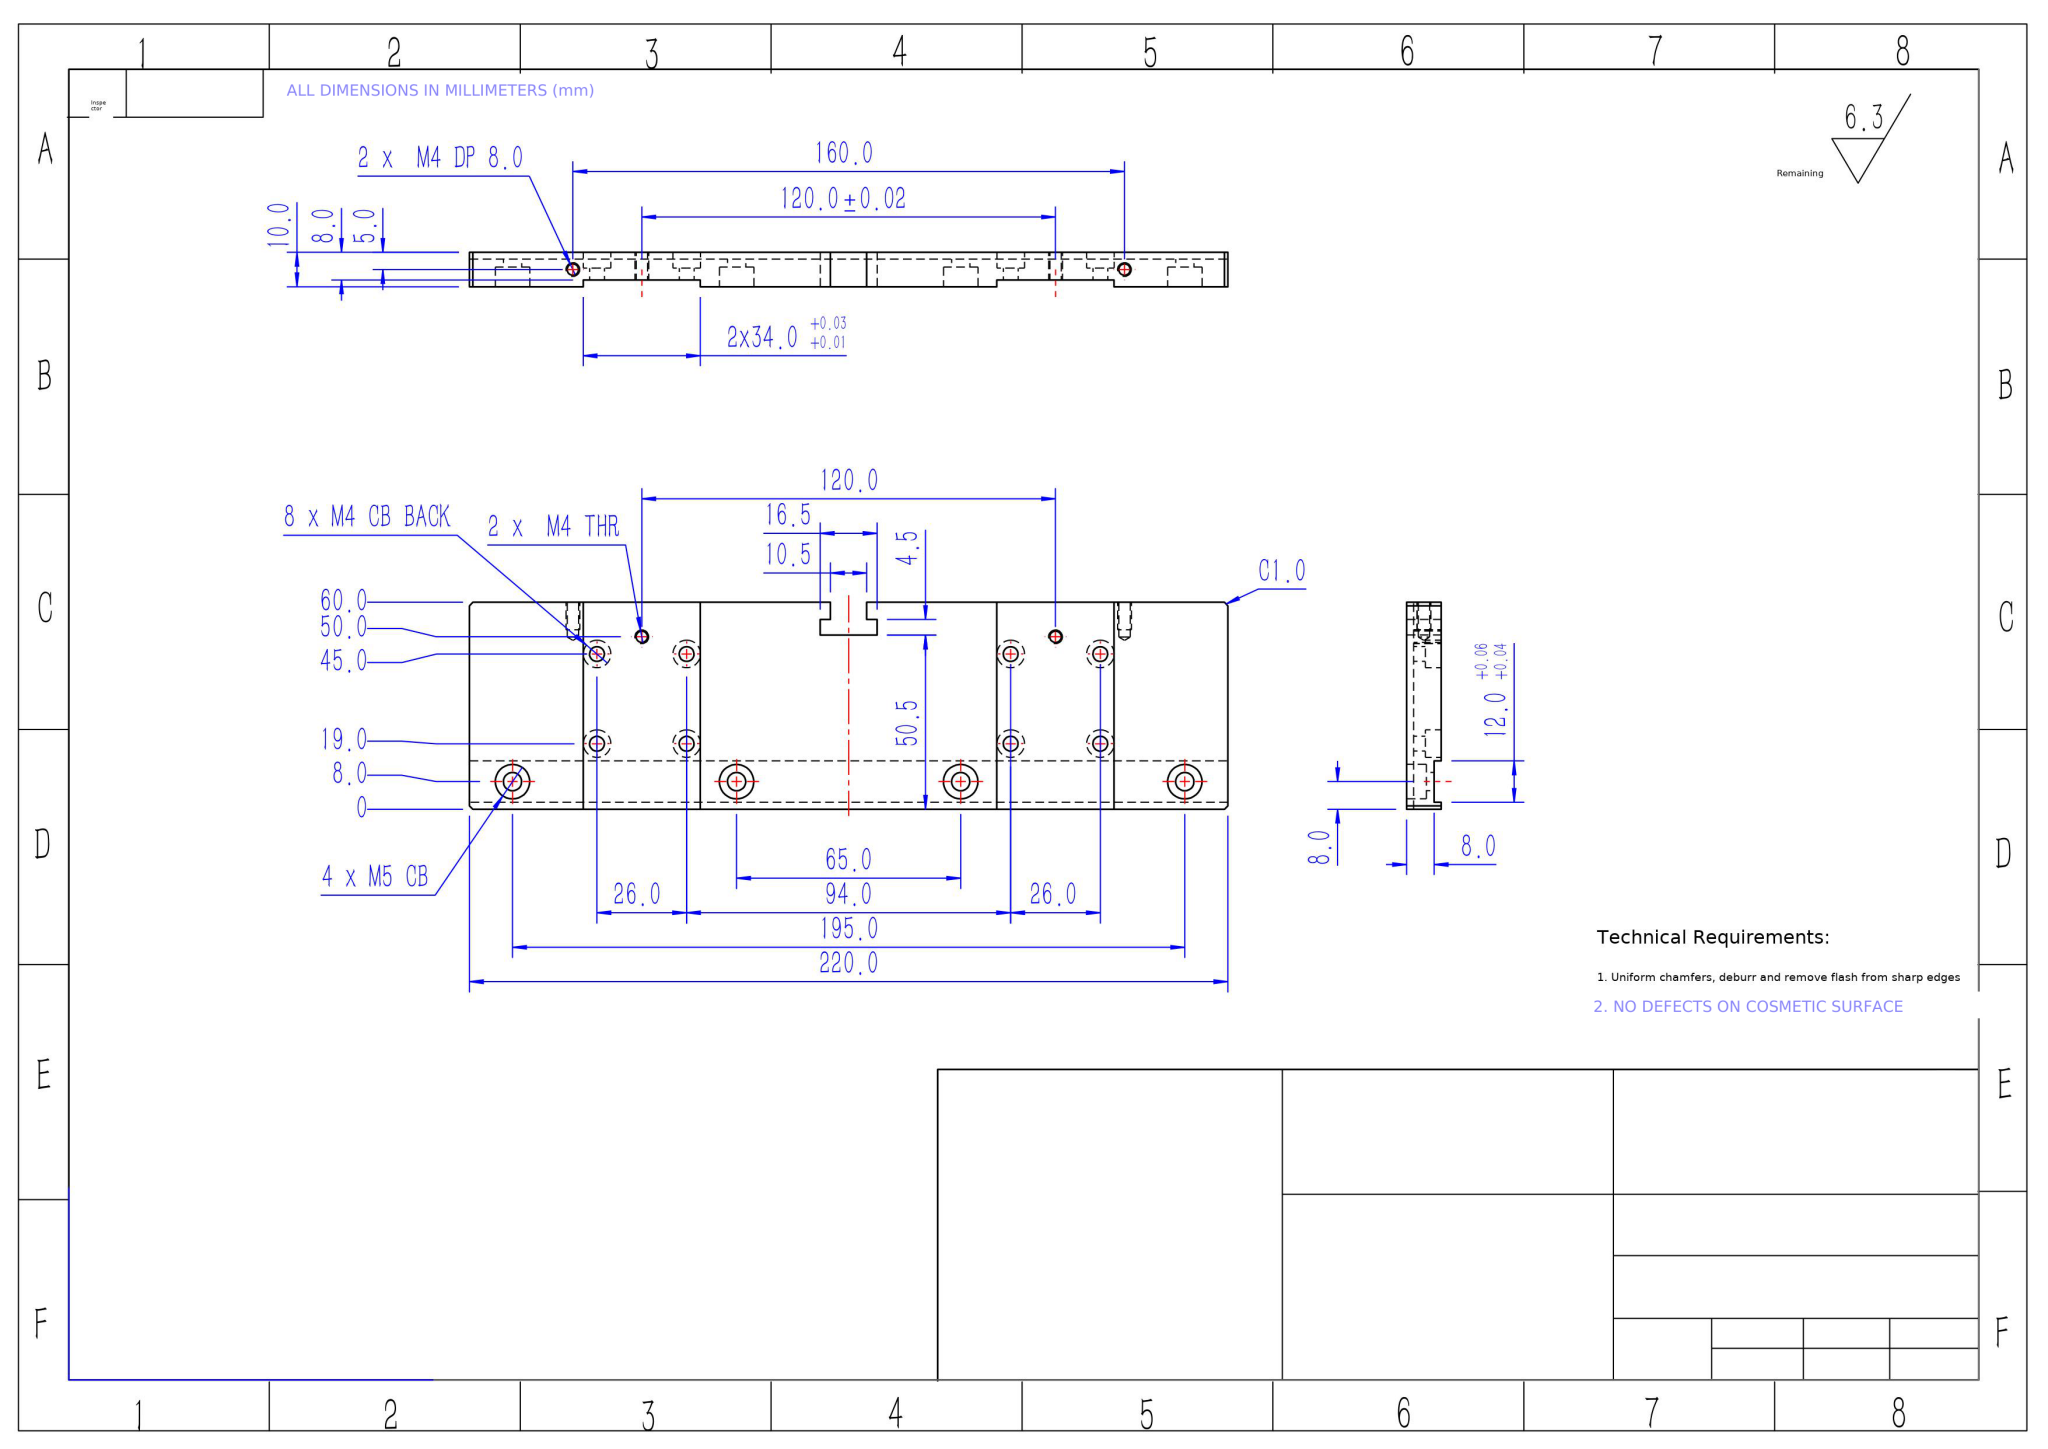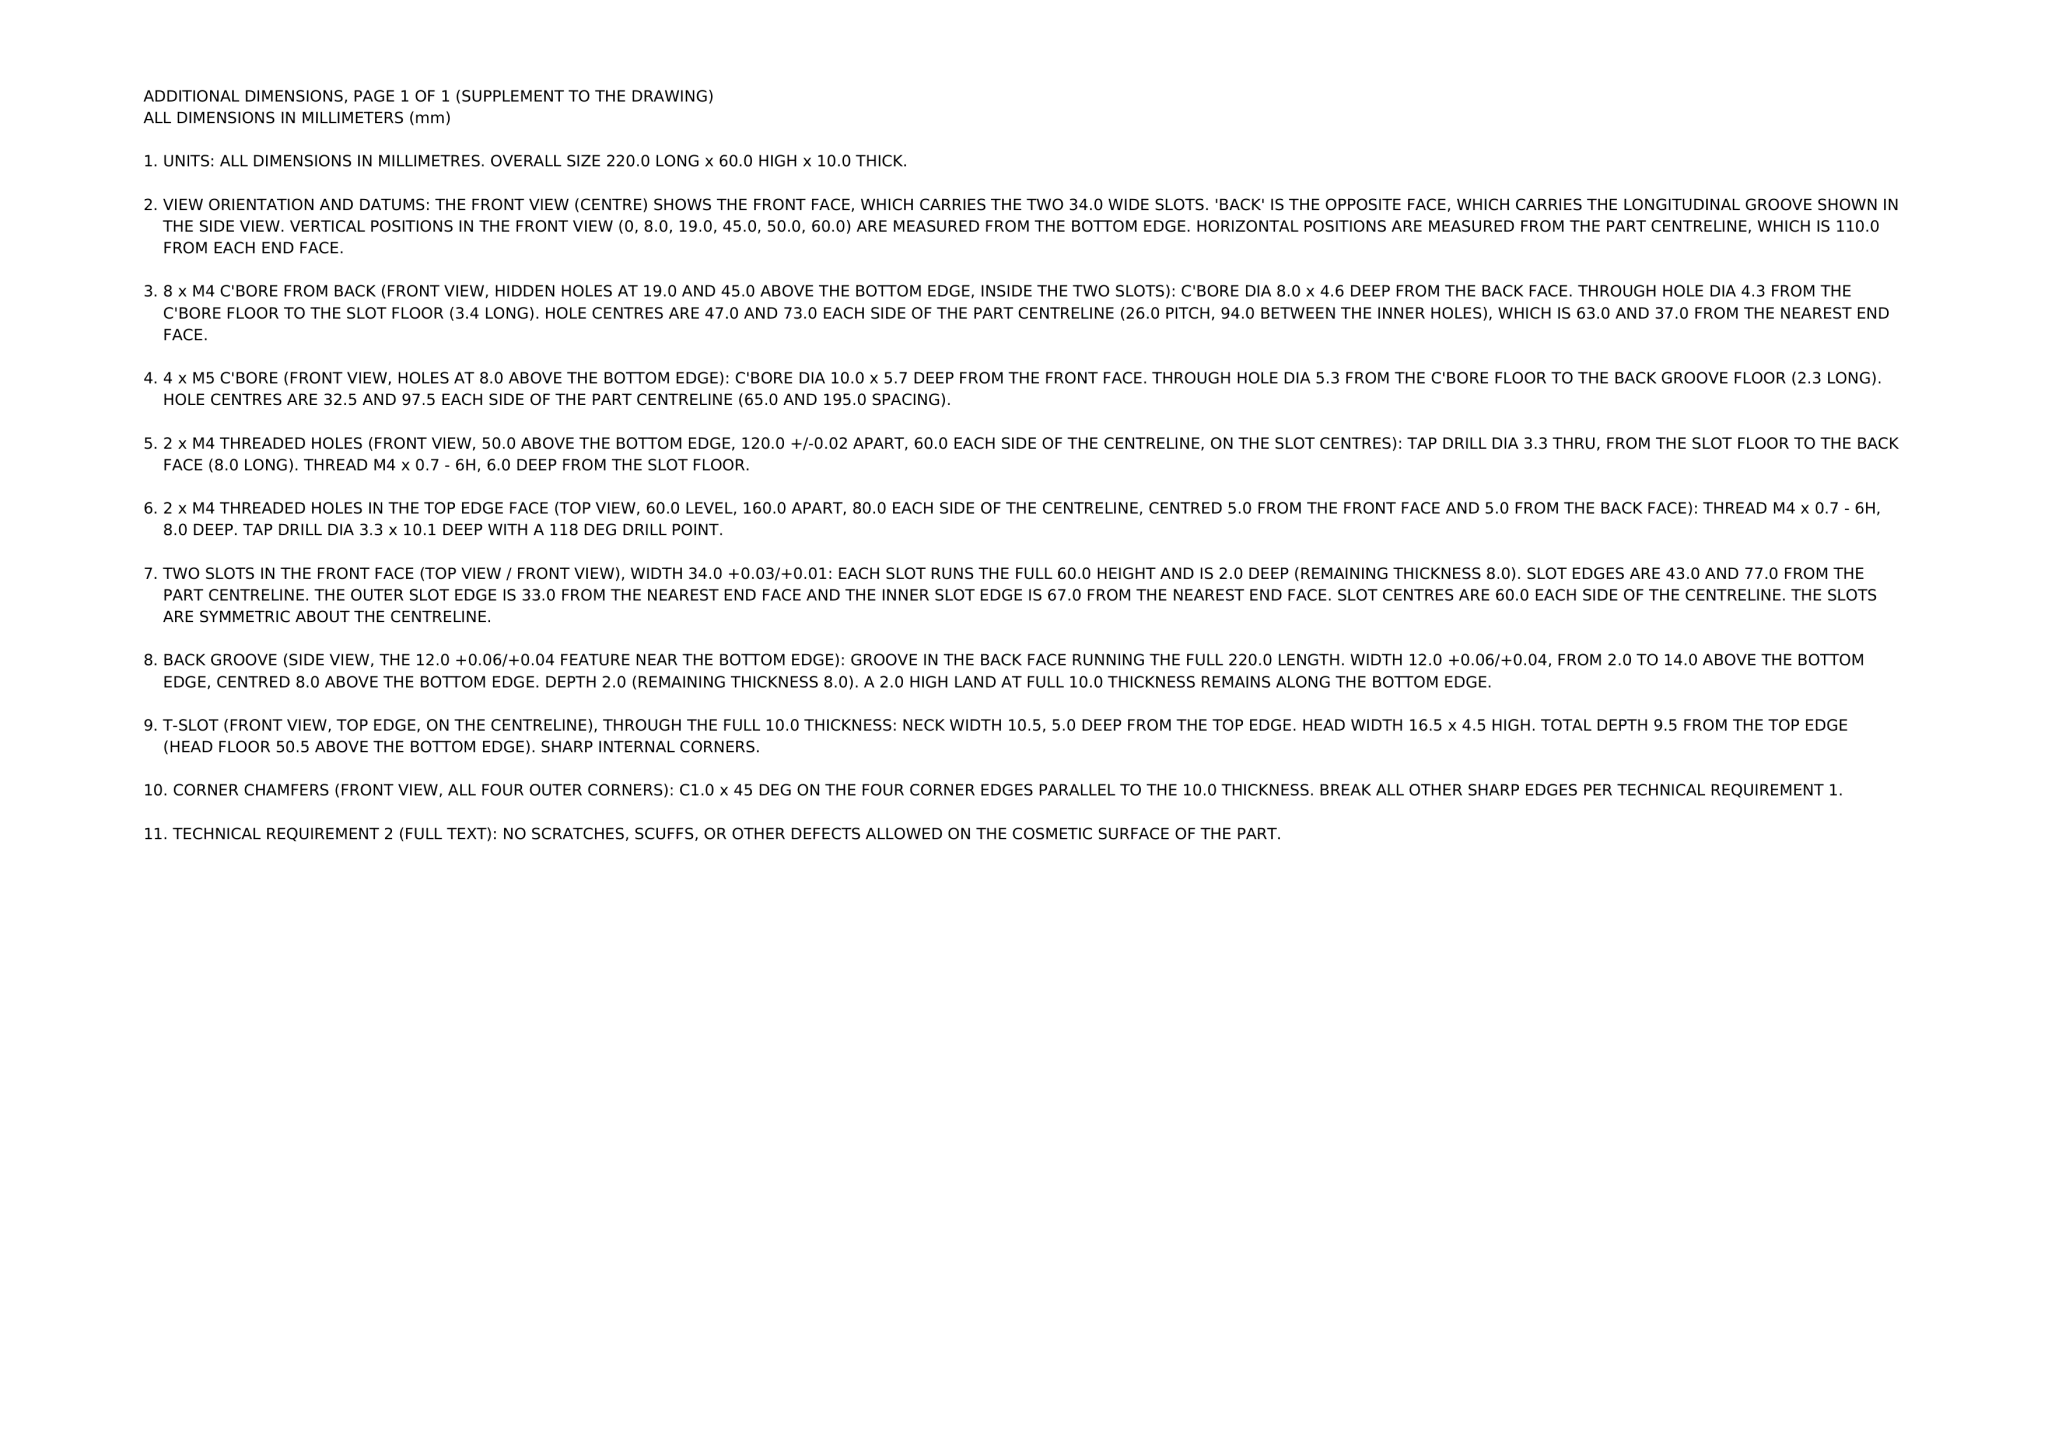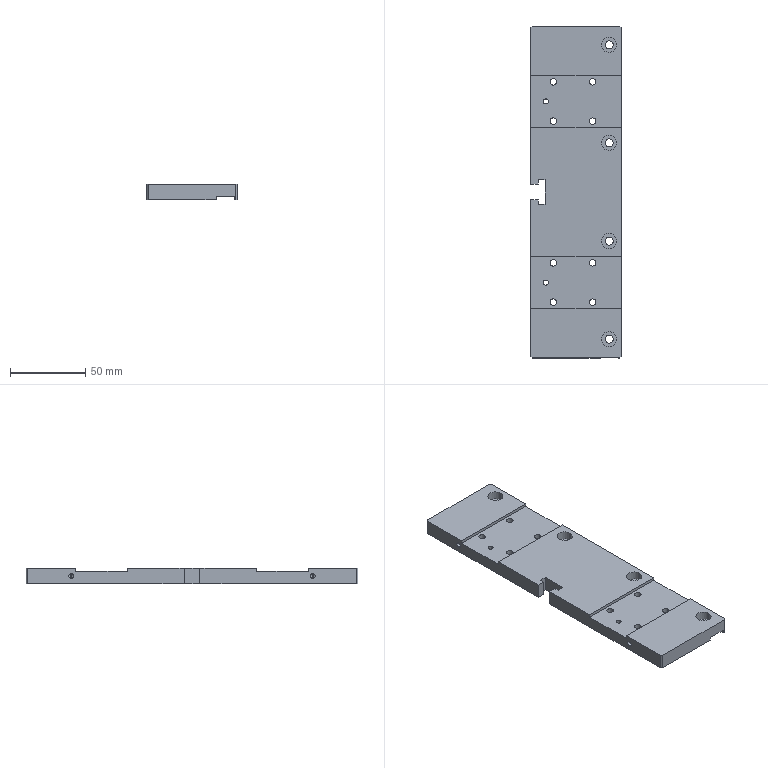Part | NX | mm | 1 solid | 102 faces | box 60 x 220 x 10 mm | volume 112719 mm3 | cylinder 56 | plane 42 | cone 4 | commonest cylinder face diameters 7.999 x16 4.3 x16 3.3 x8 10 x8 5.3 x8